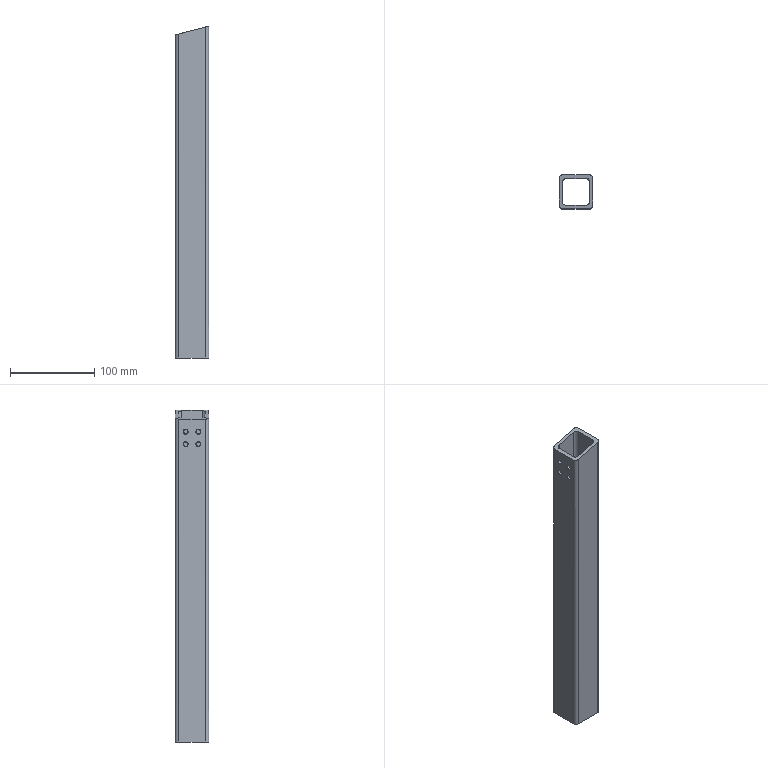Component | NX | SLANT_VERT_ROD_2_2 | 1 solid | 30 faces | volume 223744 mm3 | cylinder 12 | plane 10 | cone 8 | commonest cylinder face diameters 8 x8 5 x4